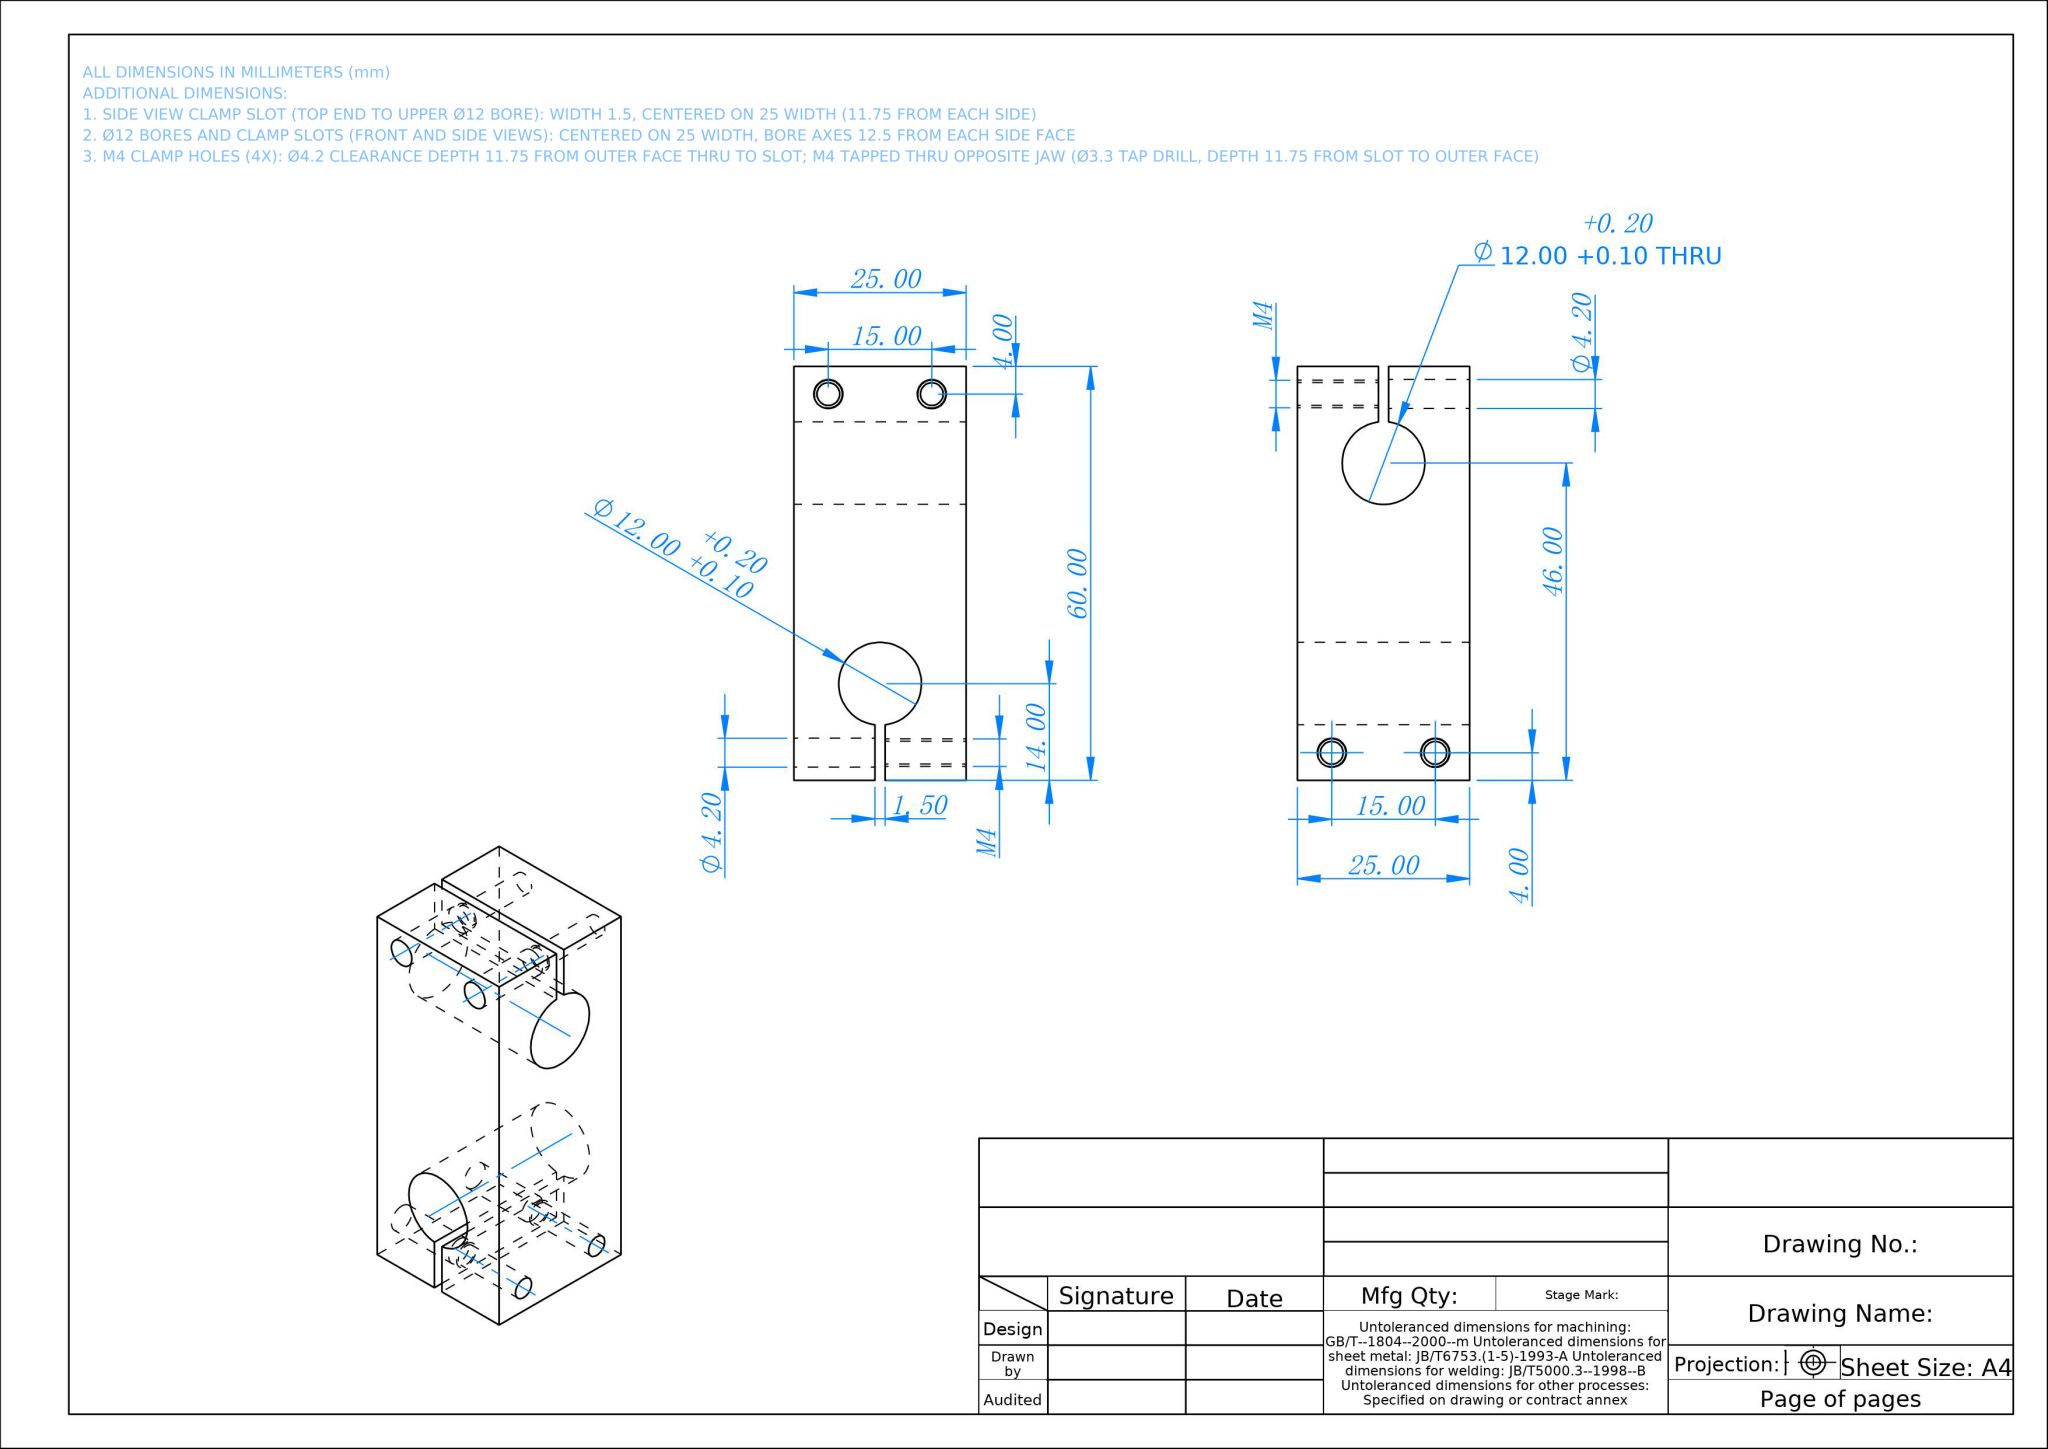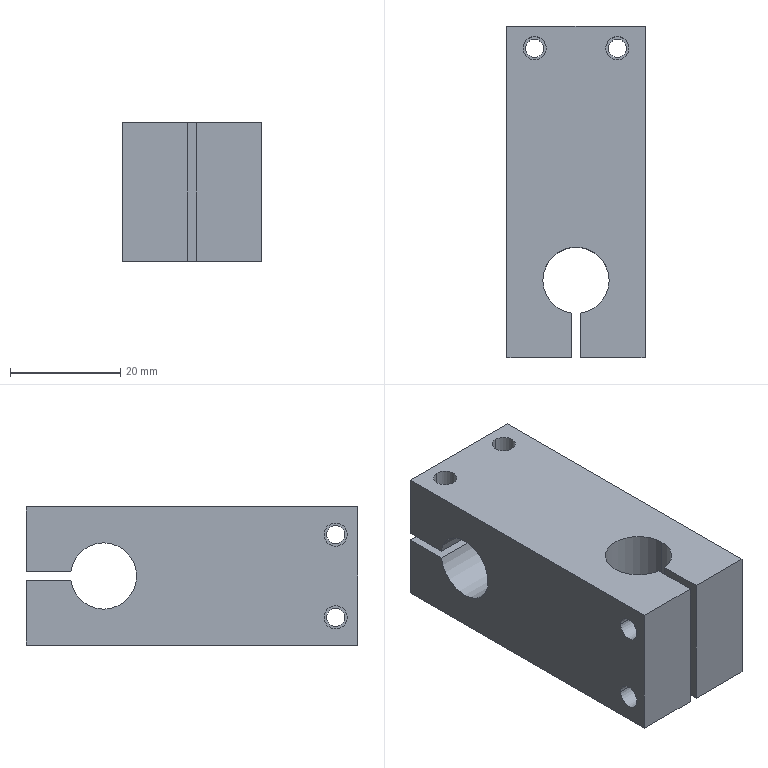Part | NX | mm | 1 solid | 32 faces | box 25 x 60 x 25 mm | volume 30191 mm3 | cylinder 20 | plane 12 | commonest cylinder face diameters 3.3 x8 4.2 x8 12 x4